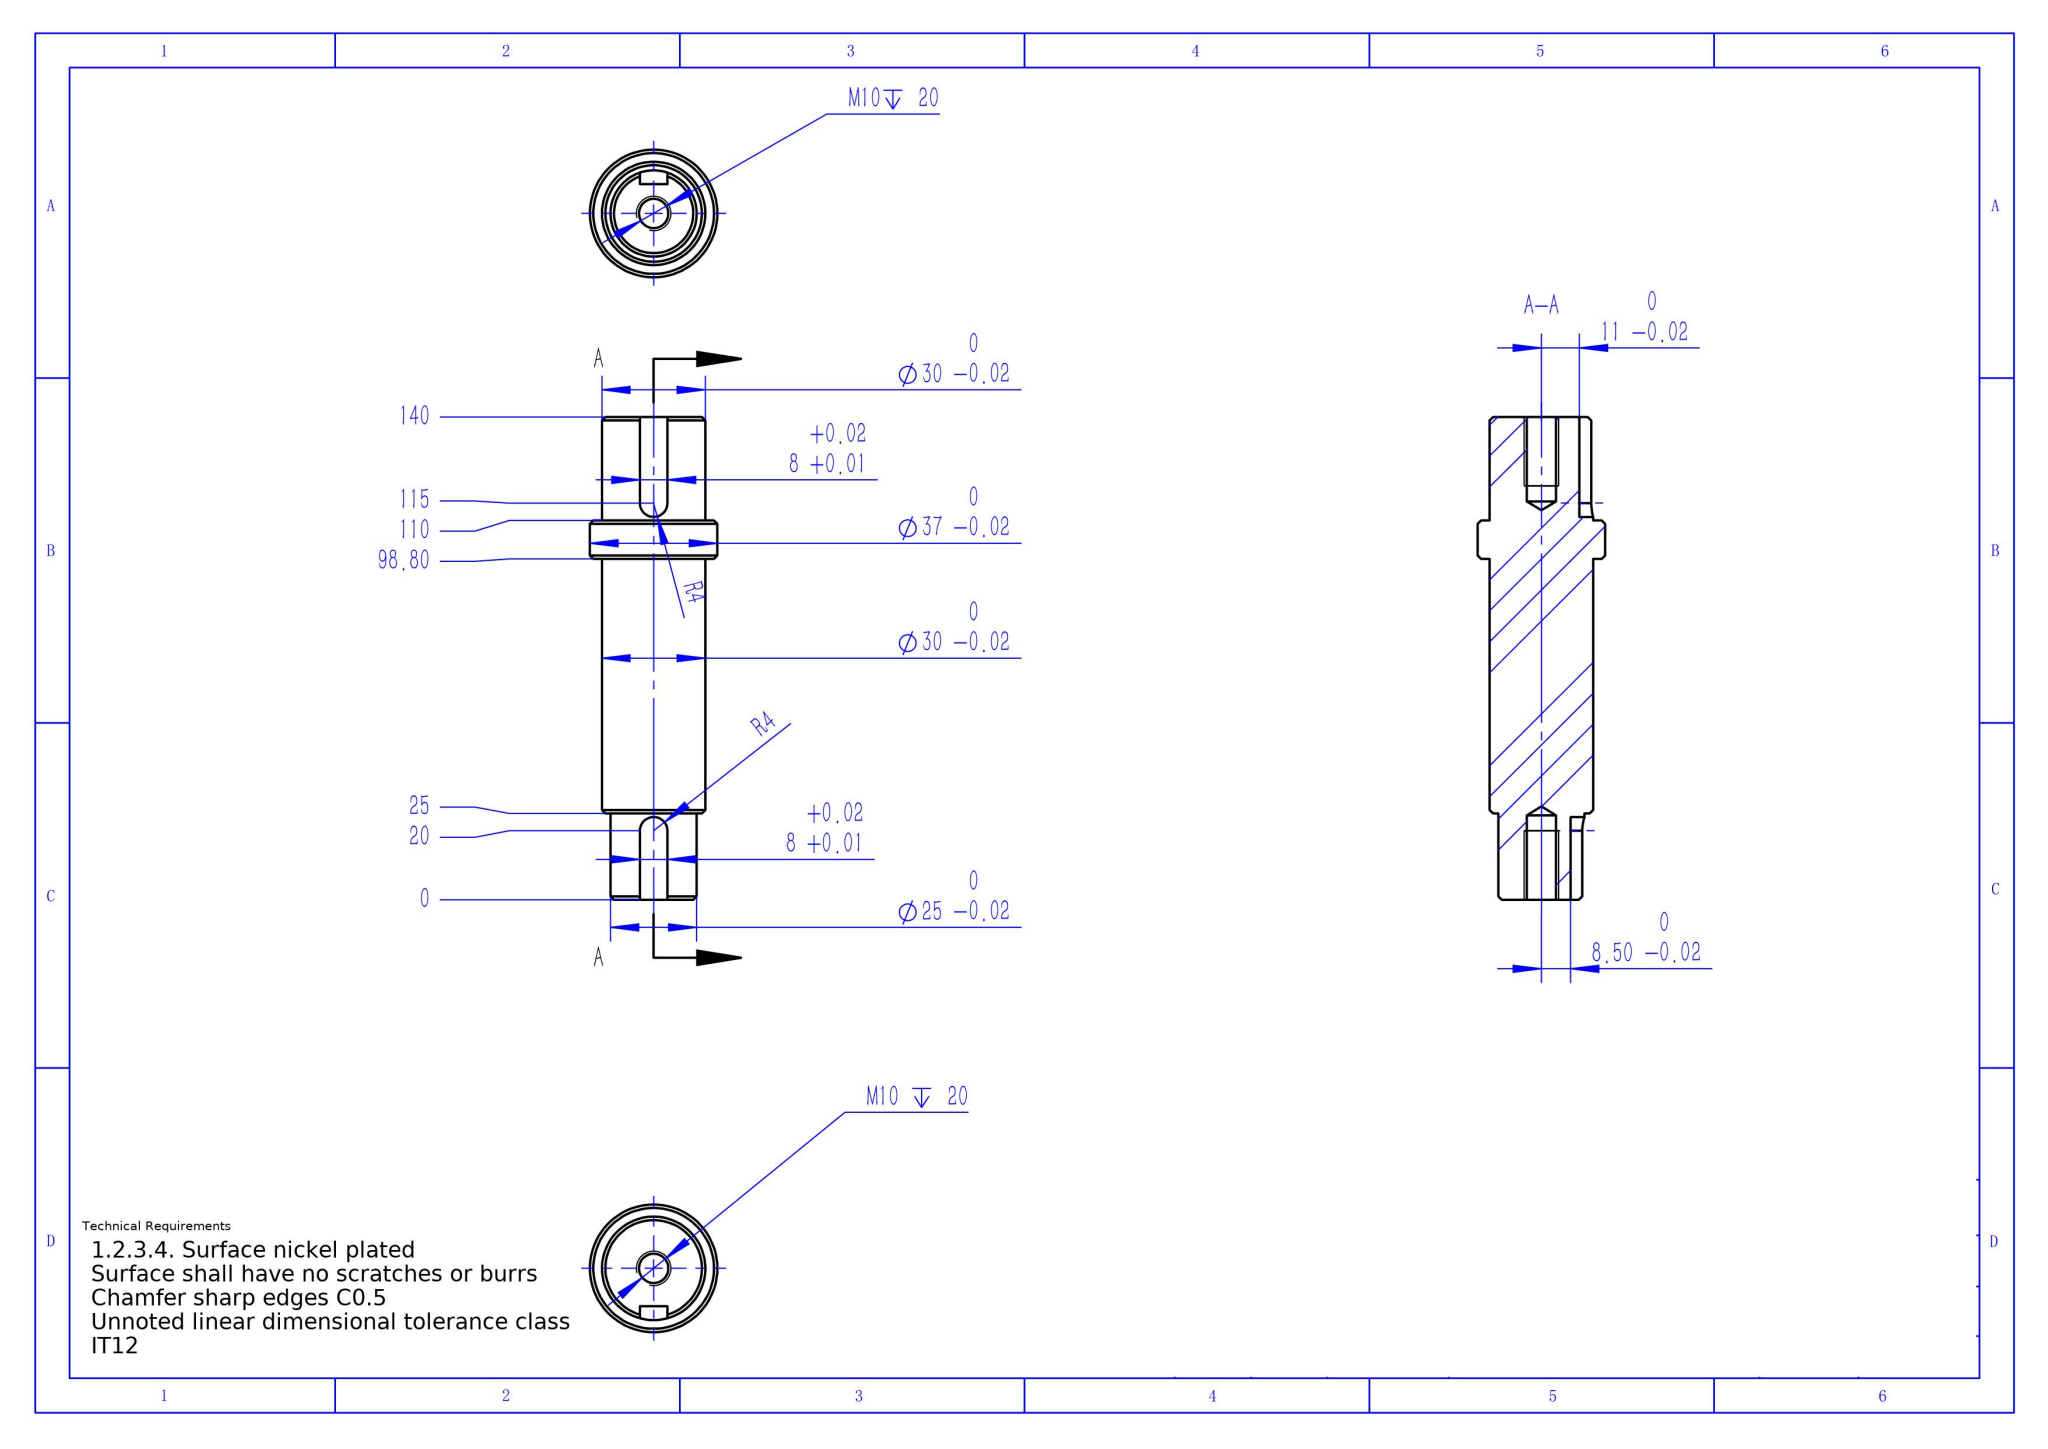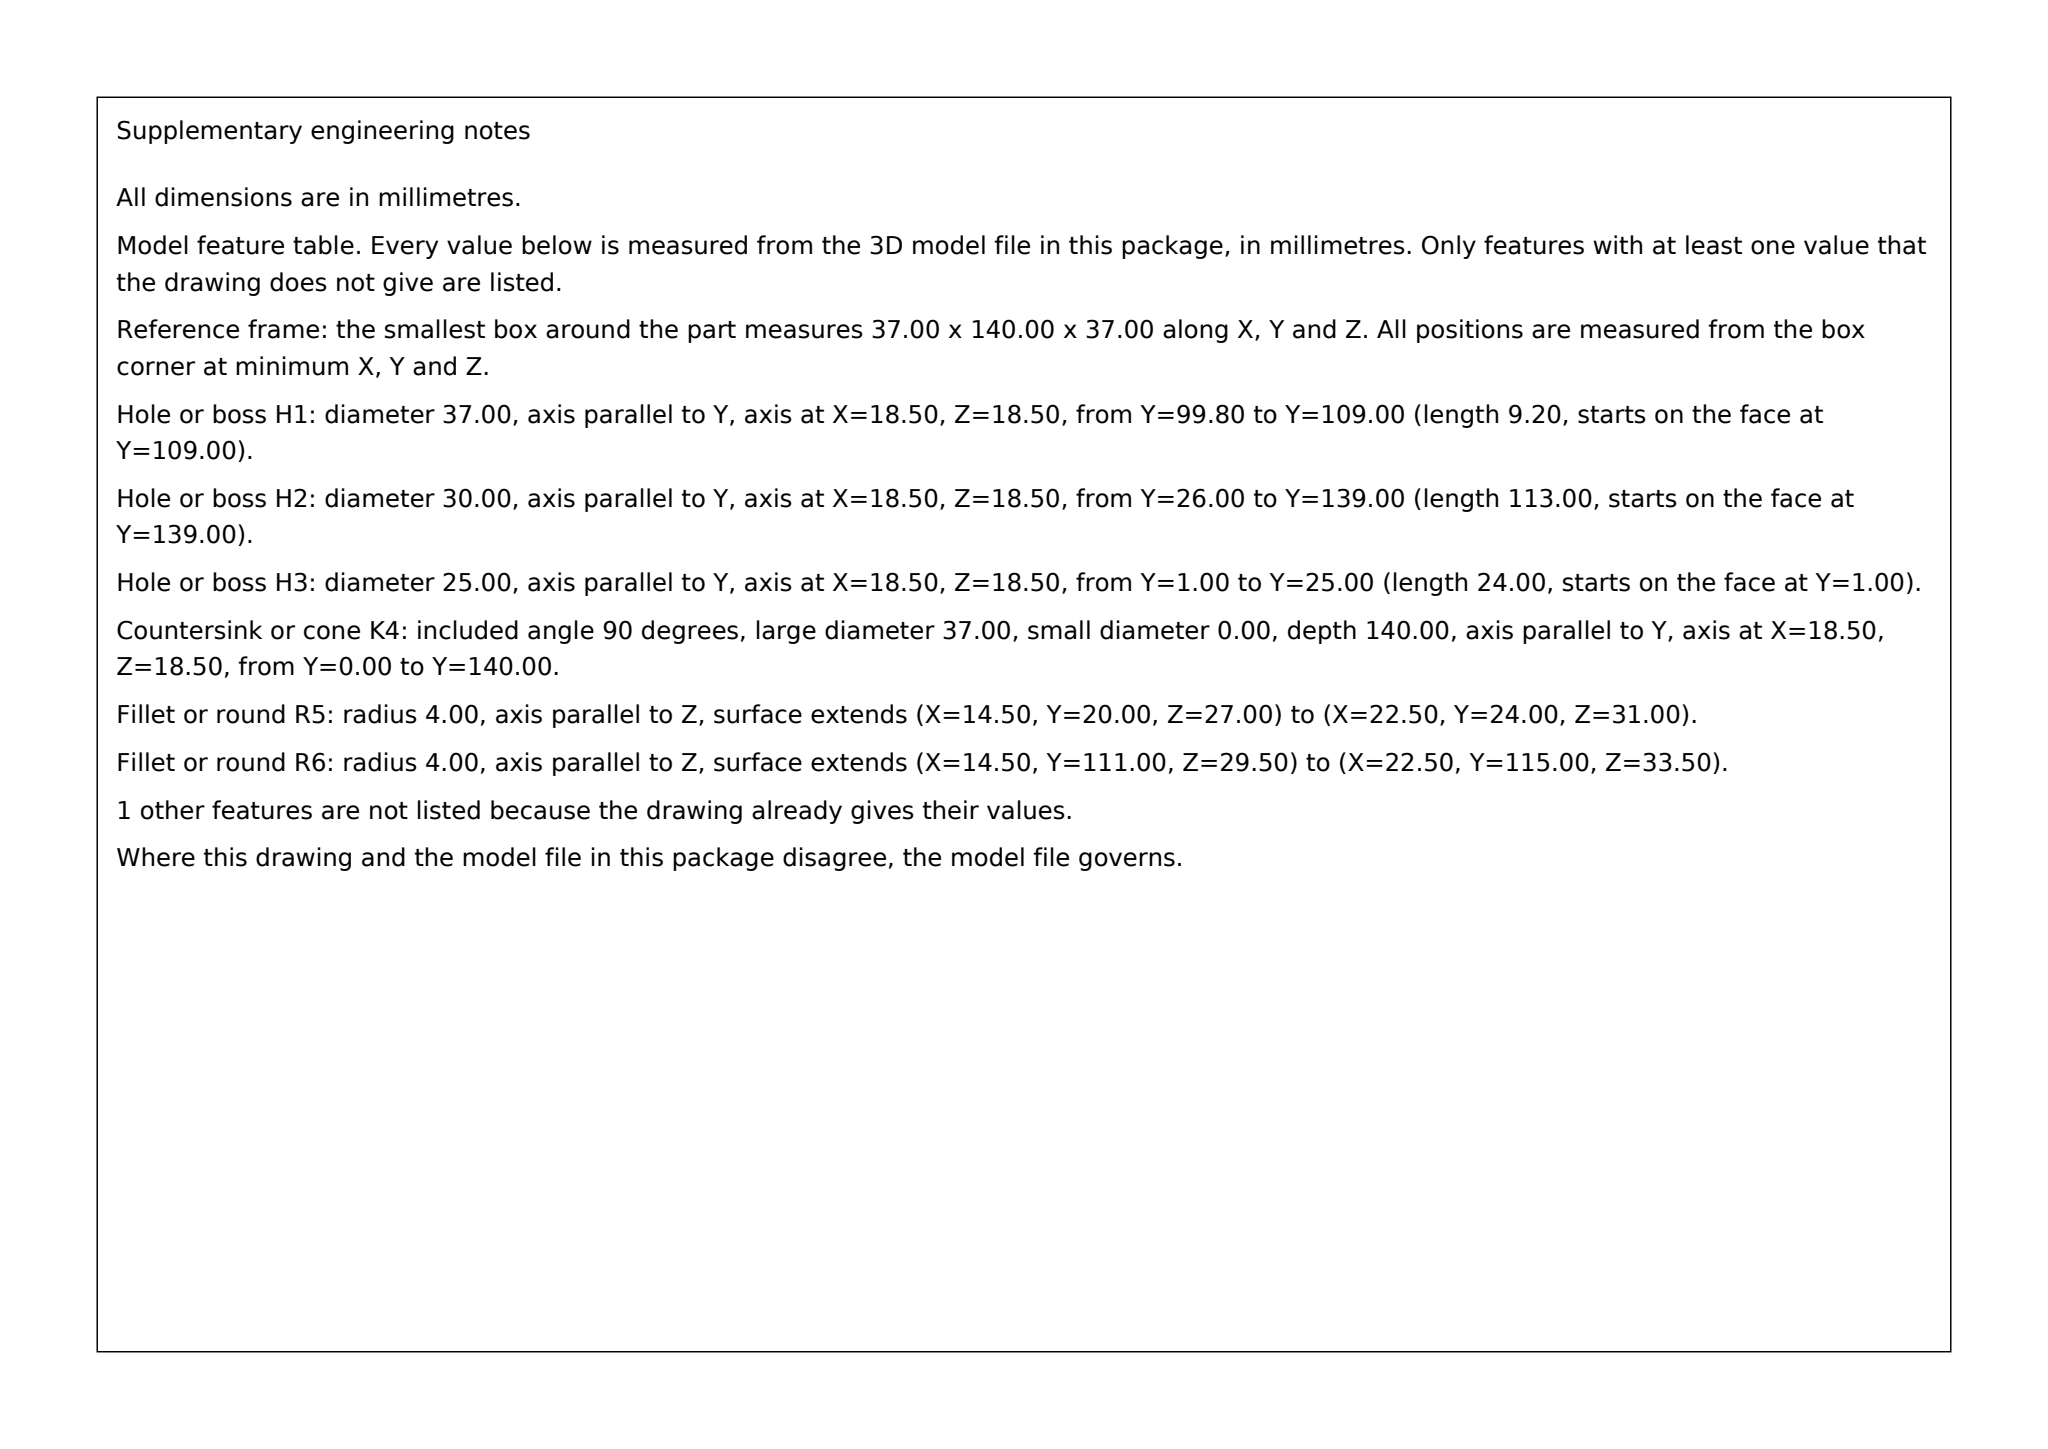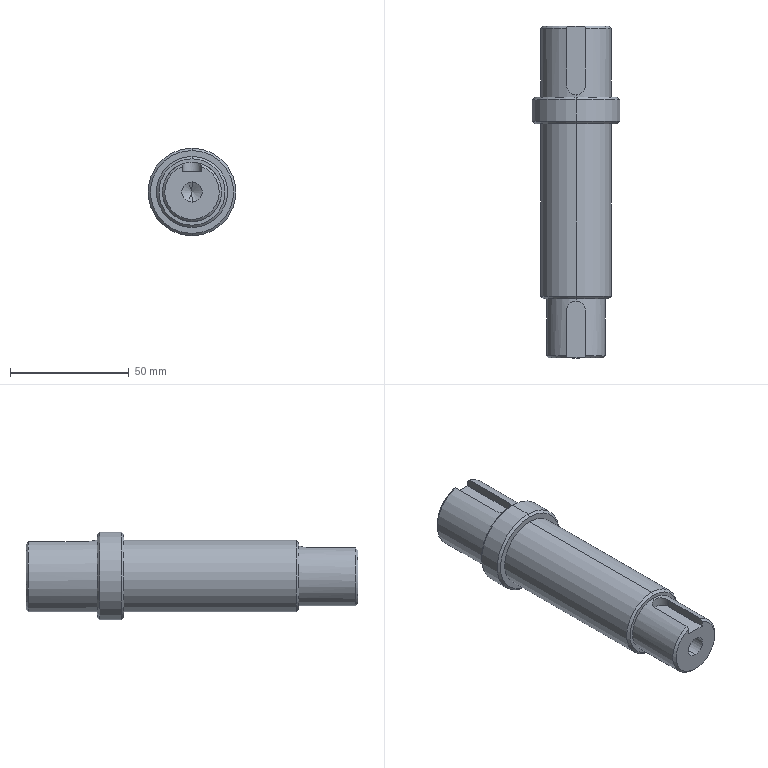Part | SolidWorks | mm | 1 solid | 38 faces | box 37 x 140 x 37 mm | volume 93010 mm3 | cylinder 14 | cone 13 | plane 11 | commonest cylinder face diameters 8.5 x4 30 x4 37 x2 25 x2 8 x2
build123d program:
from build123d import *

# Parameters (mm, degrees)
SKETCH11_R             = 20
ROUND_STEEL_40_1_DEPTH = 140
CUT_EXTRUDE1_DEPTH     = 4
M10_TAPPED_HOLE1_D     = 8.5
M10_TAPPED_HOLE1_DEPTH = 24.5
M10_TAPPED_HOLE1_TIP   = 2.554
CUT_EXTRUDE11_DEPTH    = 4
CHAMFER1_SIZE          = 1
M10_TAPPED_HOLE2_D     = 8.5
M10_TAPPED_HOLE2_DEPTH = 24.5
M10_TAPPED_HOLE2_TIP   = 2.554


with BuildPart() as part:
    # Sketch11 → Round Steel 40_1 (new body)
    with BuildSketch(Plane(origin=(0, 0, 0), x_dir=(-1, 0, 0), z_dir=(0, 1, 0))):
        Circle(SKETCH11_R)
    extrude(amount=ROUND_STEEL_40_1_DEPTH)

    # Sketch3_2 → Cut-Revolve1 (revolve, cut)
    with BuildSketch(Plane.XY, mode=Mode.PRIVATE) as cut_revolve1_sk:
        Polygon((-15, 98.8), (-18.5, 98.8), (-18.5, 110), (-15, 110), (-15, 140), (-20, 140), (-20, 0), (-12.5, 0), (-12.5, 25), (-15, 25), align=None)
    revolve(cut_revolve1_sk.sketch.rotate(Axis((0, 0, 0), (0, 1, 0)), 270), axis=Axis((0, 0, 0), (0, 1, 0)), mode=Mode.SUBTRACT)

    # Sketch3 → Cut-Extrude1 (cut)
    with BuildSketch(Plane(origin=(0, 0, 12.5), x_dir=(0, -1, 0), z_dir=(0, 0, -1))):
        with BuildLine():
            Line((0, 4), (-20, 4))
            ThreePointArc((-20, 4), (-24, 0), (-20, -4))
            Line((-20, -4), (0, -4))
            ThreePointArc((0, -4), (4, 0), (0, 4))
        make_face()
    extrude(amount=CUT_EXTRUDE1_DEPTH, mode=Mode.SUBTRACT)

    # M10 Tapped Hole1
    with Locations(Plane(origin=(0, 0, 0), x_dir=(-1, 0, 0), z_dir=(0, -1, 0))):
        with Locations((0, 0)):
            Hole(M10_TAPPED_HOLE1_D / 2, depth=M10_TAPPED_HOLE1_DEPTH)
            with Locations((0, 0, -(M10_TAPPED_HOLE1_DEPTH + M10_TAPPED_HOLE1_TIP / 2))):  # 118° drill point
                Cone(0, M10_TAPPED_HOLE1_D / 2, M10_TAPPED_HOLE1_TIP, mode=Mode.SUBTRACT)

    # Sketch31 → Cut-Extrude11 (cut)
    with BuildSketch(Plane(origin=(-0.7499, 140, 15), x_dir=(0, 1, 0), z_dir=(0, 0, -1))):
        with BuildLine():
            Line((0, 4.75), (-25, 4.75))
            ThreePointArc((-25, 4.75), (-29, 0.7499), (-25, -3.25))
            Line((-25, -3.25), (0, -3.25))
            ThreePointArc((0, -3.25), (4, 0.7499), (0, 4.75))
        make_face()
    extrude(amount=CUT_EXTRUDE11_DEPTH, mode=Mode.SUBTRACT)

    # Chamfer1
    chamfer1_edges = [part.edges().sort_by_distance(p)[0] for p in [
        (-12.335, 0, -2.027),
        (14.864, 140, -2.018),
        (0, 25, 15),
        (0, 98.8, 18.5),
        (0, 110, 18.5),
    ]]
    chamfer(chamfer1_edges, length=CHAMFER1_SIZE)

    # M10 Tapped Hole2
    with Locations(Plane(origin=(0, 140, 0), x_dir=(1, 0, 0), z_dir=(0, 1, 0))):
        with Locations((0, 0)):
            Hole(M10_TAPPED_HOLE2_D / 2, depth=M10_TAPPED_HOLE2_DEPTH)
            with Locations((0, 0, -(M10_TAPPED_HOLE2_DEPTH + M10_TAPPED_HOLE2_TIP / 2))):  # 118° drill point
                Cone(0, M10_TAPPED_HOLE2_D / 2, M10_TAPPED_HOLE2_TIP, mode=Mode.SUBTRACT)


solid = part.part